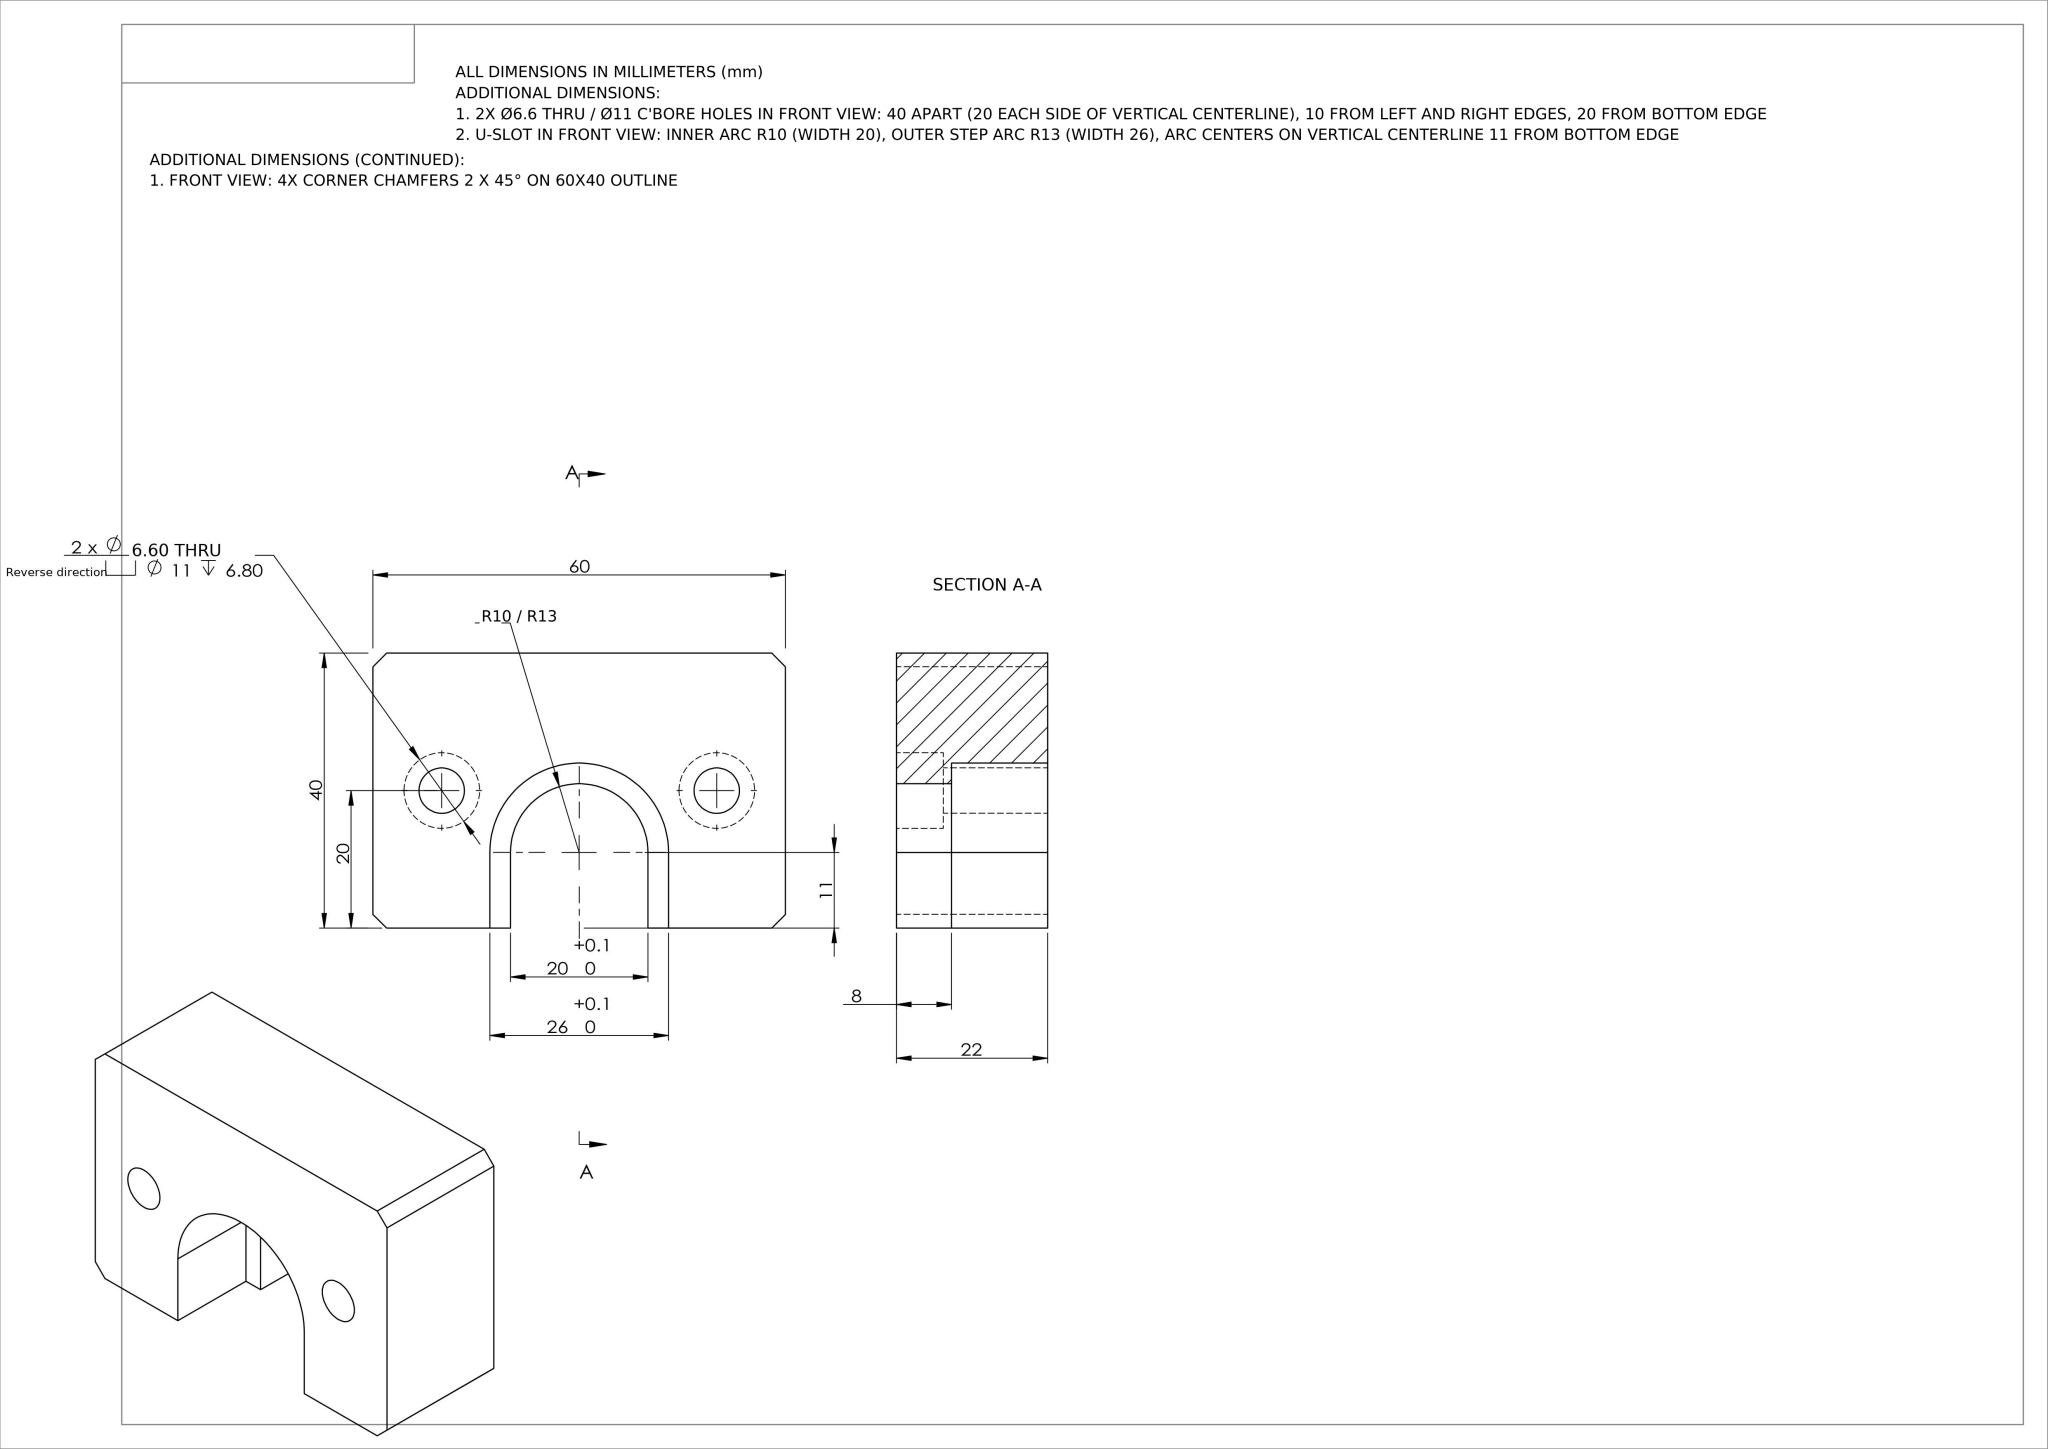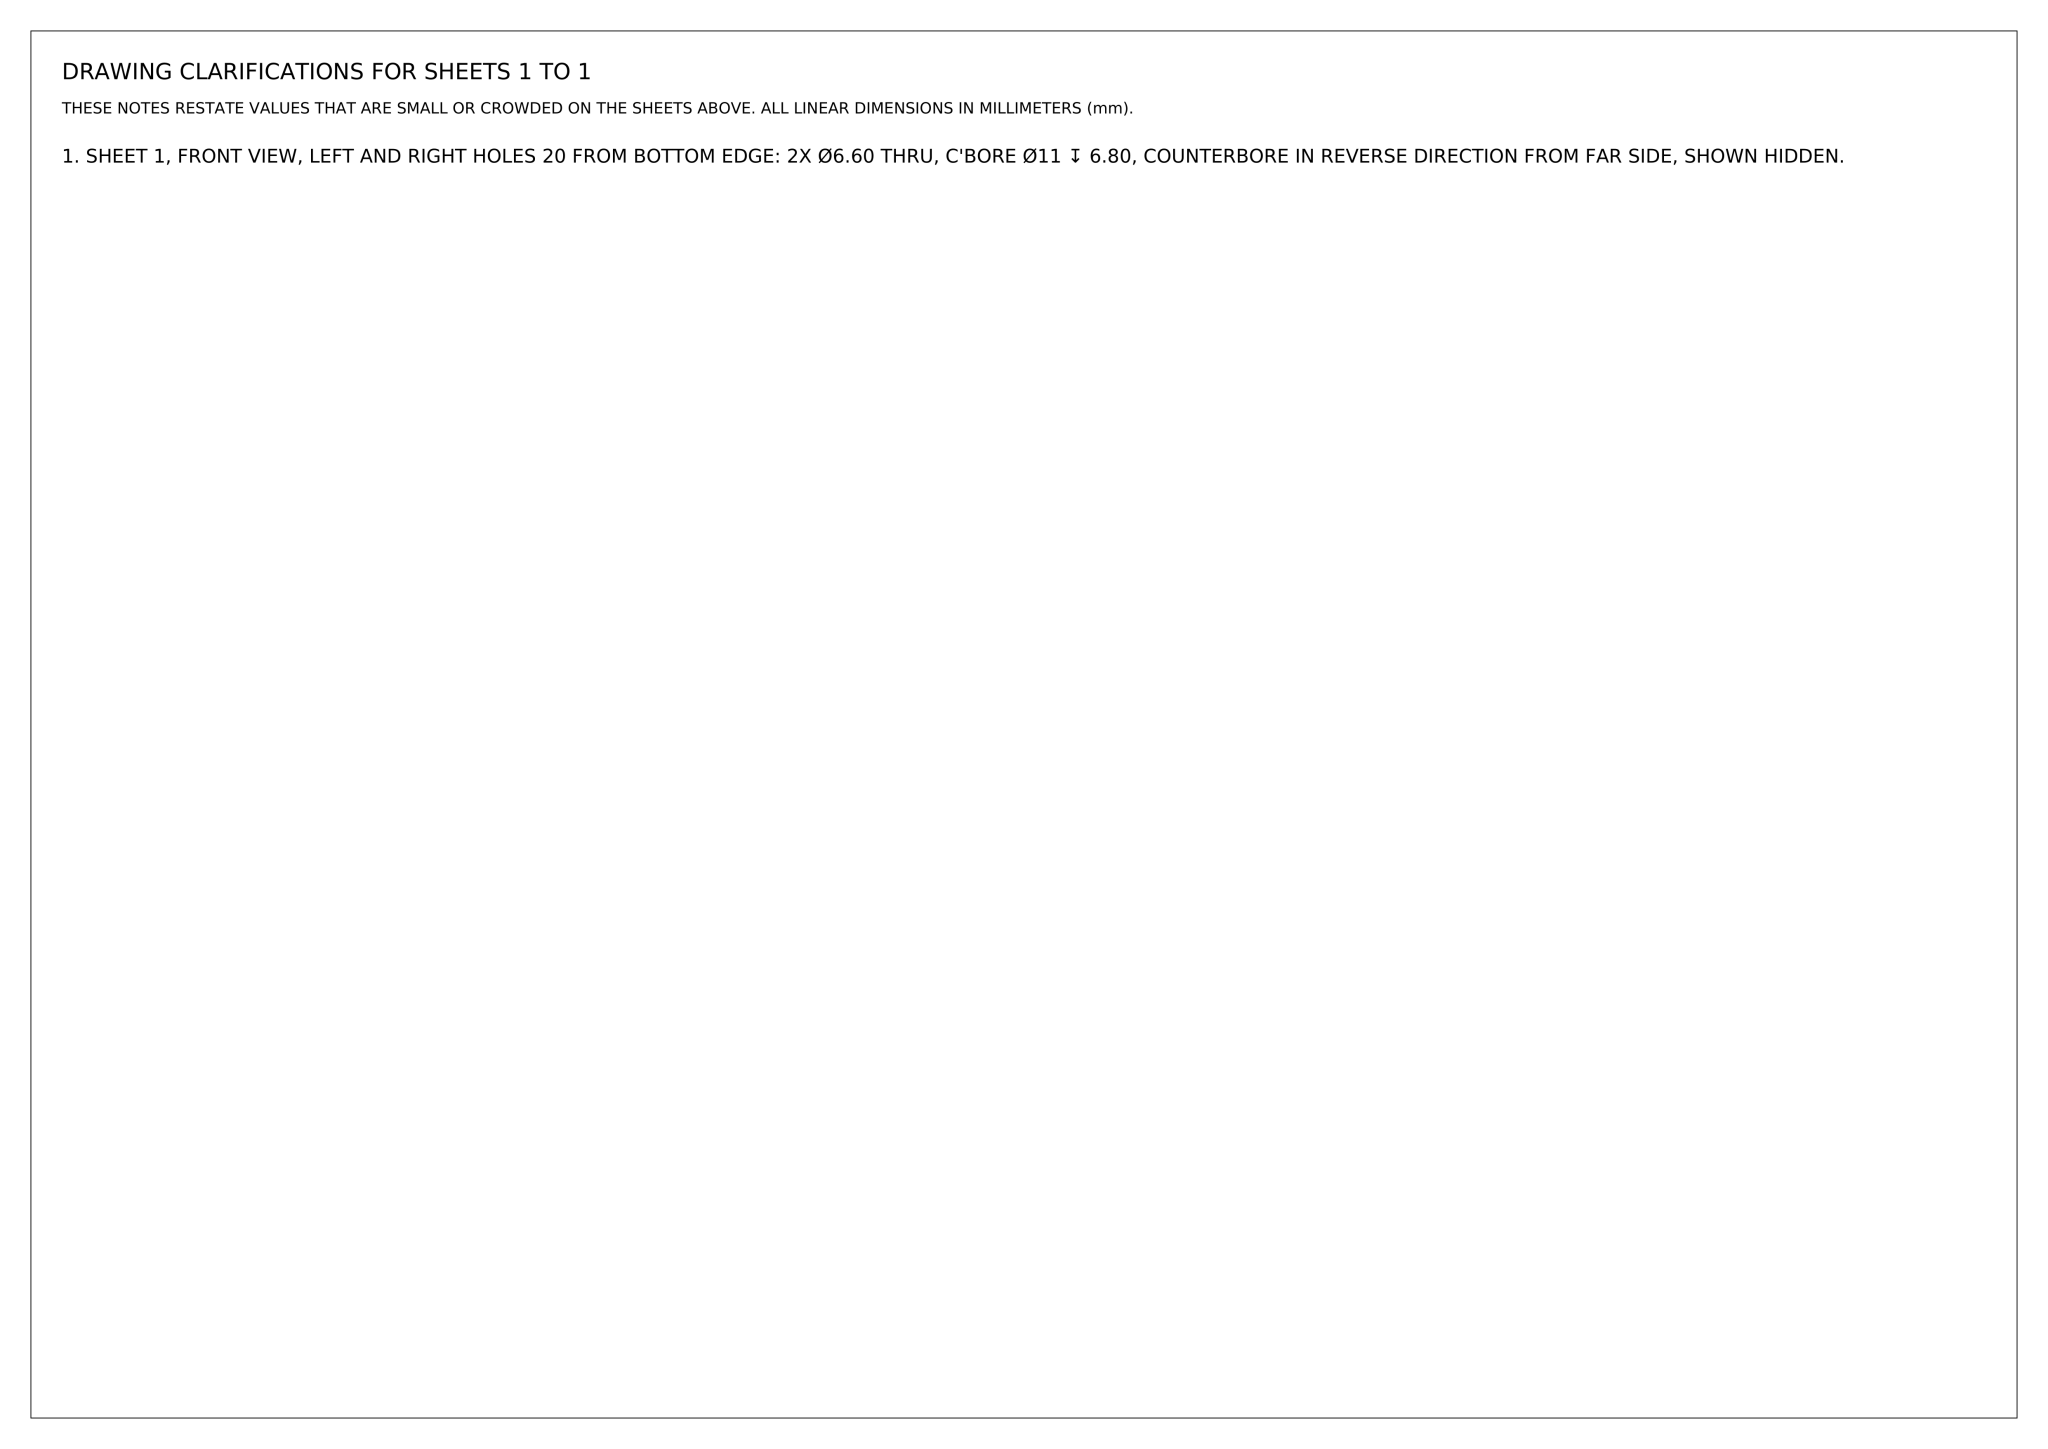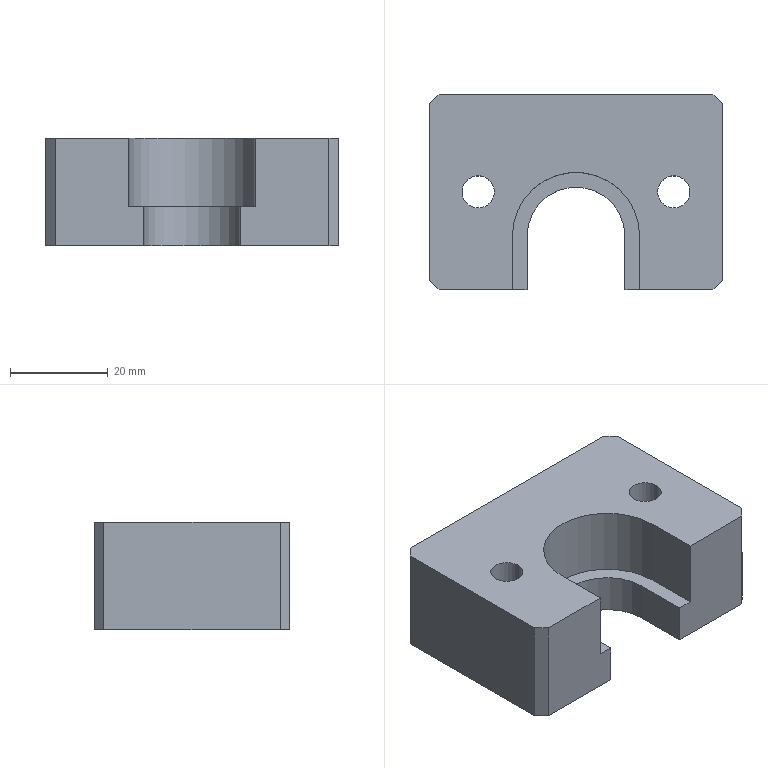Part | NX | mm | 1 solid | 28 faces | box 60 x 40 x 22 mm | volume 39554 mm3 | plane 18 | cylinder 10 | commonest cylinder face diameters 11 x4 6.6 x4 20 x1 26 x1
STEP:
#1=COLOUR_RGB('',0.6157,0.6431,0.6745);
#2=FILL_AREA_STYLE_COLOUR('',#1);
#3=FILL_AREA_STYLE('',(#2));
#4=SURFACE_STYLE_FILL_AREA(#3);
#5=SURFACE_SIDE_STYLE('',(#4));
#6=SURFACE_STYLE_USAGE(.BOTH.,#5);
#7=PRESENTATION_STYLE_ASSIGNMENT((#6));
#8=CARTESIAN_POINT('',(25.5,-0.,6.8));
#9=VERTEX_POINT('',#8);
#10=CARTESIAN_POINT('',(14.5,-0.,6.8));
#11=VERTEX_POINT('',#10);
#12=CARTESIAN_POINT('',(20.,-0.,6.8));
#13=DIRECTION('',(0.,0.,-1.));
#14=DIRECTION('',(-1.,0.,0.));
#15=AXIS2_PLACEMENT_3D('',#12,#13,#14);
#16=CIRCLE('',#15,5.5);
#17=EDGE_CURVE('',#9,#11,#16,.T.);
#18=ORIENTED_EDGE('',*,*,#17,.F.);
#19=CARTESIAN_POINT('',(25.5,-0.,0.));
#20=VERTEX_POINT('',#19);
#21=CARTESIAN_POINT('',(25.5,-0.,0.));
#22=DIRECTION('',(0.,0.,-1.));
#23=VECTOR('',#22,1000.);
#24=LINE('',#21,#23);
#25=EDGE_CURVE('',#9,#20,#24,.T.);
#26=ORIENTED_EDGE('',*,*,#25,.T.);
#27=CARTESIAN_POINT('',(14.5,-0.,0.));
#28=VERTEX_POINT('',#27);
#29=CARTESIAN_POINT('',(20.,-0.,0.));
#30=DIRECTION('',(0.,0.,-1.));
#31=DIRECTION('',(-1.,0.,0.));
#32=AXIS2_PLACEMENT_3D('',#29,#30,#31);
#33=CIRCLE('',#32,5.5);
#34=EDGE_CURVE('',#20,#28,#33,.T.);
#35=ORIENTED_EDGE('',*,*,#34,.T.);
#36=CARTESIAN_POINT('',(14.5,-0.,0.));
#37=DIRECTION('',(0.,0.,-1.));
#38=VECTOR('',#37,1000.);
#39=LINE('',#36,#38);
#40=EDGE_CURVE('',#11,#28,#39,.T.);
#41=ORIENTED_EDGE('',*,*,#40,.F.);
#42=EDGE_LOOP('',(#18,#26,#35,#41));
#43=FACE_OUTER_BOUND('',#42,.T.);
#44=CARTESIAN_POINT('',(20.,-0.,0.));
#45=DIRECTION('',(0.,0.,-1.));
#46=DIRECTION('',(-1.,0.,0.));
#47=AXIS2_PLACEMENT_3D('',#44,#45,#46);
#48=CYLINDRICAL_SURFACE('',#47,5.5);
#49=ADVANCED_FACE('',(#43),#48,.F.);
#50=CARTESIAN_POINT('',(23.3,-0.,22.));
#51=VERTEX_POINT('',#50);
#52=CARTESIAN_POINT('',(16.7,-0.,22.));
#53=VERTEX_POINT('',#52);
#54=CARTESIAN_POINT('',(20.,-0.,22.));
#55=DIRECTION('',(0.,0.,-1.));
#56=DIRECTION('',(-1.,0.,0.));
#57=AXIS2_PLACEMENT_3D('',#54,#55,#56);
#58=CIRCLE('',#57,3.3);
#59=EDGE_CURVE('',#51,#53,#58,.T.);
#60=ORIENTED_EDGE('',*,*,#59,.F.);
#61=CARTESIAN_POINT('',(23.3,-0.,6.8));
#62=VERTEX_POINT('',#61);
#63=CARTESIAN_POINT('',(23.3,-0.,0.));
#64=DIRECTION('',(0.,0.,-1.));
#65=VECTOR('',#64,1000.);
#66=LINE('',#63,#65);
#67=EDGE_CURVE('',#51,#62,#66,.T.);
#68=ORIENTED_EDGE('',*,*,#67,.T.);
#69=CARTESIAN_POINT('',(16.7,-0.,6.8));
#70=VERTEX_POINT('',#69);
#71=CARTESIAN_POINT('',(20.,-0.,6.8));
#72=DIRECTION('',(0.,0.,-1.));
#73=DIRECTION('',(-1.,0.,0.));
#74=AXIS2_PLACEMENT_3D('',#71,#72,#73);
#75=CIRCLE('',#74,3.3);
#76=EDGE_CURVE('',#62,#70,#75,.T.);
#77=ORIENTED_EDGE('',*,*,#76,.T.);
#78=CARTESIAN_POINT('',(16.7,-0.,0.));
#79=DIRECTION('',(0.,0.,-1.));
#80=VECTOR('',#79,1000.);
#81=LINE('',#78,#80);
#82=EDGE_CURVE('',#53,#70,#81,.T.);
#83=ORIENTED_EDGE('',*,*,#82,.F.);
#84=EDGE_LOOP('',(#60,#68,#77,#83));
#85=FACE_OUTER_BOUND('',#84,.T.);
#86=CARTESIAN_POINT('',(20.,-0.,0.));
#87=DIRECTION('',(0.,0.,-1.));
#88=DIRECTION('',(-1.,0.,0.));
#89=AXIS2_PLACEMENT_3D('',#86,#87,#88);
#90=CYLINDRICAL_SURFACE('',#89,3.3);
#91=ADVANCED_FACE('',(#85),#90,.F.);
#92=CARTESIAN_POINT('',(-14.5,-0.,6.8));
#93=VERTEX_POINT('',#92);
#94=CARTESIAN_POINT('',(-25.5,-0.,6.8));
#95=VERTEX_POINT('',#94);
#96=CARTESIAN_POINT('',(-20.,-0.,6.8));
#97=DIRECTION('',(0.,0.,-1.));
#98=DIRECTION('',(-1.,0.,0.));
#99=AXIS2_PLACEMENT_3D('',#96,#97,#98);
#100=CIRCLE('',#99,5.5);
#101=EDGE_CURVE('',#93,#95,#100,.T.);
#102=ORIENTED_EDGE('',*,*,#101,.F.);
#103=CARTESIAN_POINT('',(-14.5,-0.,0.));
#104=VERTEX_POINT('',#103);
#105=CARTESIAN_POINT('',(-14.5,-0.,0.));
#106=DIRECTION('',(0.,0.,-1.));
#107=VECTOR('',#106,1000.);
#108=LINE('',#105,#107);
#109=EDGE_CURVE('',#93,#104,#108,.T.);
#110=ORIENTED_EDGE('',*,*,#109,.T.);
#111=CARTESIAN_POINT('',(-25.5,-0.,0.));
#112=VERTEX_POINT('',#111);
#113=CARTESIAN_POINT('',(-20.,-0.,0.));
#114=DIRECTION('',(0.,0.,-1.));
#115=DIRECTION('',(-1.,0.,0.));
#116=AXIS2_PLACEMENT_3D('',#113,#114,#115);
#117=CIRCLE('',#116,5.5);
#118=EDGE_CURVE('',#104,#112,#117,.T.);
#119=ORIENTED_EDGE('',*,*,#118,.T.);
#120=CARTESIAN_POINT('',(-25.5,-0.,0.));
#121=DIRECTION('',(0.,0.,-1.));
#122=VECTOR('',#121,1000.);
#123=LINE('',#120,#122);
#124=EDGE_CURVE('',#95,#112,#123,.T.);
#125=ORIENTED_EDGE('',*,*,#124,.F.);
#126=EDGE_LOOP('',(#102,#110,#119,#125));
#127=FACE_OUTER_BOUND('',#126,.T.);
#128=CARTESIAN_POINT('',(-20.,-0.,0.));
#129=DIRECTION('',(0.,0.,-1.));
#130=DIRECTION('',(-1.,0.,0.));
#131=AXIS2_PLACEMENT_3D('',#128,#129,#130);
#132=CYLINDRICAL_SURFACE('',#131,5.5);
#133=ADVANCED_FACE('',(#127),#132,.F.);
#134=CARTESIAN_POINT('',(-16.7,-0.,22.));
#135=VERTEX_POINT('',#134);
#136=CARTESIAN_POINT('',(-23.3,-0.,22.));
#137=VERTEX_POINT('',#136);
#138=CARTESIAN_POINT('',(-20.,-0.,22.));
#139=DIRECTION('',(0.,0.,-1.));
#140=DIRECTION('',(-1.,0.,0.));
#141=AXIS2_PLACEMENT_3D('',#138,#139,#140);
#142=CIRCLE('',#141,3.3);
#143=EDGE_CURVE('',#135,#137,#142,.T.);
#144=ORIENTED_EDGE('',*,*,#143,.F.);
#145=CARTESIAN_POINT('',(-16.7,-0.,6.8));
#146=VERTEX_POINT('',#145);
#147=CARTESIAN_POINT('',(-16.7,-0.,0.));
#148=DIRECTION('',(0.,0.,-1.));
#149=VECTOR('',#148,1000.);
#150=LINE('',#147,#149);
#151=EDGE_CURVE('',#135,#146,#150,.T.);
#152=ORIENTED_EDGE('',*,*,#151,.T.);
#153=CARTESIAN_POINT('',(-23.3,-0.,6.8));
#154=VERTEX_POINT('',#153);
#155=CARTESIAN_POINT('',(-20.,-0.,6.8));
#156=DIRECTION('',(0.,0.,-1.));
#157=DIRECTION('',(-1.,0.,0.));
#158=AXIS2_PLACEMENT_3D('',#155,#156,#157);
#159=CIRCLE('',#158,3.3);
#160=EDGE_CURVE('',#146,#154,#159,.T.);
#161=ORIENTED_EDGE('',*,*,#160,.T.);
#162=CARTESIAN_POINT('',(-23.3,-0.,0.));
#163=DIRECTION('',(0.,0.,-1.));
#164=VECTOR('',#163,1000.);
#165=LINE('',#162,#164);
#166=EDGE_CURVE('',#137,#154,#165,.T.);
#167=ORIENTED_EDGE('',*,*,#166,.F.);
#168=EDGE_LOOP('',(#144,#152,#161,#167));
#169=FACE_OUTER_BOUND('',#168,.T.);
#170=CARTESIAN_POINT('',(-20.,-0.,0.));
#171=DIRECTION('',(0.,0.,-1.));
#172=DIRECTION('',(-1.,0.,0.));
#173=AXIS2_PLACEMENT_3D('',#170,#171,#172);
#174=CYLINDRICAL_SURFACE('',#173,3.3);
#175=ADVANCED_FACE('',(#169),#174,.F.);
#176=CARTESIAN_POINT('',(-10.,-20.,8.));
#177=VERTEX_POINT('',#176);
#178=CARTESIAN_POINT('',(-10.,-9.,8.));
#179=VERTEX_POINT('',#178);
#180=CARTESIAN_POINT('',(-10.,-20.,8.));
#181=DIRECTION('',(0.,1.,0.));
#182=VECTOR('',#181,1000.);
#183=LINE('',#180,#182);
#184=EDGE_CURVE('',#177,#179,#183,.T.);
#185=ORIENTED_EDGE('',*,*,#184,.F.);
#186=CARTESIAN_POINT('',(-10.,-20.,0.));
#187=VERTEX_POINT('',#186);
#188=CARTESIAN_POINT('',(-10.,-20.,0.));
#189=DIRECTION('',(0.,0.,1.));
#190=VECTOR('',#189,1000.);
#191=LINE('',#188,#190);
#192=EDGE_CURVE('',#187,#177,#191,.T.);
#193=ORIENTED_EDGE('',*,*,#192,.F.);
#194=CARTESIAN_POINT('',(-10.,-9.,0.));
#195=VERTEX_POINT('',#194);
#196=CARTESIAN_POINT('',(-10.,-20.,0.));
#197=DIRECTION('',(0.,-1.,0.));
#198=VECTOR('',#197,1000.);
#199=LINE('',#196,#198);
#200=EDGE_CURVE('',#195,#187,#199,.T.);
#201=ORIENTED_EDGE('',*,*,#200,.F.);
#202=CARTESIAN_POINT('',(-10.,-9.,0.));
#203=DIRECTION('',(0.,0.,1.));
#204=VECTOR('',#203,1000.);
#205=LINE('',#202,#204);
#206=EDGE_CURVE('',#195,#179,#205,.T.);
#207=ORIENTED_EDGE('',*,*,#206,.T.);
#208=EDGE_LOOP('',(#185,#193,#201,#207));
#209=FACE_OUTER_BOUND('',#208,.T.);
#210=CARTESIAN_POINT('',(-10.,-20.,0.));
#211=DIRECTION('',(-1.,0.,0.));
#212=DIRECTION('',(0.,0.,1.));
#213=AXIS2_PLACEMENT_3D('',#210,#211,#212);
#214=PLANE('',#213);
#215=ADVANCED_FACE('',(#209),#214,.F.);
#216=CARTESIAN_POINT('',(10.,-9.,8.));
#217=VERTEX_POINT('',#216);
#218=CARTESIAN_POINT('',(0.,-9.,8.));
#219=DIRECTION('',(0.,0.,-1.));
#220=DIRECTION('',(1.,0.,0.));
#221=AXIS2_PLACEMENT_3D('',#218,#219,#220);
#222=CIRCLE('',#221,10.);
#223=EDGE_CURVE('',#179,#217,#222,.T.);
#224=ORIENTED_EDGE('',*,*,#223,.F.);
#225=ORIENTED_EDGE('',*,*,#206,.F.);
#226=CARTESIAN_POINT('',(10.,-9.,0.));
#227=VERTEX_POINT('',#226);
#228=CARTESIAN_POINT('',(0.,-9.,0.));
#229=DIRECTION('',(0.,0.,1.));
#230=DIRECTION('',(1.,0.,0.));
#231=AXIS2_PLACEMENT_3D('',#228,#229,#230);
#232=CIRCLE('',#231,10.);
#233=EDGE_CURVE('',#227,#195,#232,.T.);
#234=ORIENTED_EDGE('',*,*,#233,.F.);
#235=CARTESIAN_POINT('',(10.,-9.,0.));
#236=DIRECTION('',(0.,0.,1.));
#237=VECTOR('',#236,1000.);
#238=LINE('',#235,#237);
#239=EDGE_CURVE('',#227,#217,#238,.T.);
#240=ORIENTED_EDGE('',*,*,#239,.T.);
#241=EDGE_LOOP('',(#224,#225,#234,#240));
#242=FACE_OUTER_BOUND('',#241,.T.);
#243=CARTESIAN_POINT('',(0.,-9.,0.));
#244=DIRECTION('',(0.,0.,1.));
#245=DIRECTION('',(1.,0.,0.));
#246=AXIS2_PLACEMENT_3D('',#243,#244,#245);
#247=CYLINDRICAL_SURFACE('',#246,10.);
#248=ADVANCED_FACE('',(#242),#247,.F.);
#249=CARTESIAN_POINT('',(10.,-20.,8.));
#250=VERTEX_POINT('',#249);
#251=CARTESIAN_POINT('',(10.,-20.,8.));
#252=DIRECTION('',(0.,-1.,0.));
#253=VECTOR('',#252,1000.);
#254=LINE('',#251,#253);
#255=EDGE_CURVE('',#217,#250,#254,.T.);
#256=ORIENTED_EDGE('',*,*,#255,.F.);
#257=ORIENTED_EDGE('',*,*,#239,.F.);
#258=CARTESIAN_POINT('',(10.,-20.,0.));
#259=VERTEX_POINT('',#258);
#260=CARTESIAN_POINT('',(10.,-20.,0.));
#261=DIRECTION('',(0.,1.,0.));
#262=VECTOR('',#261,1000.);
#263=LINE('',#260,#262);
#264=EDGE_CURVE('',#259,#227,#263,.T.);
#265=ORIENTED_EDGE('',*,*,#264,.F.);
#266=CARTESIAN_POINT('',(10.,-20.,0.));
#267=DIRECTION('',(0.,0.,1.));
#268=VECTOR('',#267,1000.);
#269=LINE('',#266,#268);
#270=EDGE_CURVE('',#259,#250,#269,.T.);
#271=ORIENTED_EDGE('',*,*,#270,.T.);
#272=EDGE_LOOP('',(#256,#257,#265,#271));
#273=FACE_OUTER_BOUND('',#272,.T.);
#274=CARTESIAN_POINT('',(10.,-20.,0.));
#275=DIRECTION('',(1.,0.,0.));
#276=DIRECTION('',(0.,0.,-1.));
#277=AXIS2_PLACEMENT_3D('',#274,#275,#276);
#278=PLANE('',#277);
#279=ADVANCED_FACE('',(#273),#278,.F.);
#280=CARTESIAN_POINT('',(-28.,-20.,22.));
#281=VERTEX_POINT('',#280);
#282=CARTESIAN_POINT('',(-13.,-20.,22.));
#283=VERTEX_POINT('',#282);
#284=CARTESIAN_POINT('',(-30.,-20.,22.));
#285=DIRECTION('',(1.,0.,0.));
#286=VECTOR('',#285,1000.);
#287=LINE('',#284,#286);
#288=EDGE_CURVE('',#281,#283,#287,.T.);
#289=ORIENTED_EDGE('',*,*,#288,.F.);
#290=CARTESIAN_POINT('',(-28.,-20.,0.));
#291=VERTEX_POINT('',#290);
#292=CARTESIAN_POINT('',(-28.,-20.,22.));
#293=DIRECTION('',(0.,0.,-1.));
#294=VECTOR('',#293,1000.);
#295=LINE('',#292,#294);
#296=EDGE_CURVE('',#281,#291,#295,.T.);
#297=ORIENTED_EDGE('',*,*,#296,.T.);
#298=CARTESIAN_POINT('',(-30.,-20.,0.));
#299=DIRECTION('',(1.,0.,0.));
#300=VECTOR('',#299,1000.);
#301=LINE('',#298,#300);
#302=EDGE_CURVE('',#291,#187,#301,.T.);
#303=ORIENTED_EDGE('',*,*,#302,.T.);
#304=ORIENTED_EDGE('',*,*,#192,.T.);
#305=CARTESIAN_POINT('',(-13.,-20.,8.));
#306=VERTEX_POINT('',#305);
#307=CARTESIAN_POINT('',(-13.,-20.,8.));
#308=DIRECTION('',(1.,0.,0.));
#309=VECTOR('',#308,1000.);
#310=LINE('',#307,#309);
#311=EDGE_CURVE('',#306,#177,#310,.T.);
#312=ORIENTED_EDGE('',*,*,#311,.F.);
#313=CARTESIAN_POINT('',(-13.,-20.,8.));
#314=DIRECTION('',(0.,0.,1.));
#315=VECTOR('',#314,1000.);
#316=LINE('',#313,#315);
#317=EDGE_CURVE('',#306,#283,#316,.T.);
#318=ORIENTED_EDGE('',*,*,#317,.T.);
#319=EDGE_LOOP('',(#289,#297,#303,#304,#312,#318));
#320=FACE_OUTER_BOUND('',#319,.T.);
#321=CARTESIAN_POINT('',(-30.,-20.,22.));
#322=DIRECTION('',(0.,1.,0.));
#323=DIRECTION('',(0.,0.,1.));
#324=AXIS2_PLACEMENT_3D('',#321,#322,#323);
#325=PLANE('',#324);
#326=ADVANCED_FACE('',(#320),#325,.F.);
#327=CARTESIAN_POINT('',(30.,-18.,22.));
#328=VERTEX_POINT('',#327);
#329=CARTESIAN_POINT('',(30.,18.,22.));
#330=VERTEX_POINT('',#329);
#331=CARTESIAN_POINT('',(30.,-20.,22.));
#332=DIRECTION('',(0.,1.,0.));
#333=VECTOR('',#332,1000.);
#334=LINE('',#331,#333);
#335=EDGE_CURVE('',#328,#330,#334,.T.);
#336=ORIENTED_EDGE('',*,*,#335,.F.);
#337=CARTESIAN_POINT('',(30.,-18.,0.));
#338=VERTEX_POINT('',#337);
#339=CARTESIAN_POINT('',(30.,-18.,22.));
#340=DIRECTION('',(0.,0.,-1.));
#341=VECTOR('',#340,1000.);
#342=LINE('',#339,#341);
#343=EDGE_CURVE('',#328,#338,#342,.T.);
#344=ORIENTED_EDGE('',*,*,#343,.T.);
#345=CARTESIAN_POINT('',(30.,18.,0.));
#346=VERTEX_POINT('',#345);
#347=CARTESIAN_POINT('',(30.,-20.,0.));
#348=DIRECTION('',(0.,1.,0.));
#349=VECTOR('',#348,1000.);
#350=LINE('',#347,#349);
#351=EDGE_CURVE('',#338,#346,#350,.T.);
#352=ORIENTED_EDGE('',*,*,#351,.T.);
#353=CARTESIAN_POINT('',(30.,18.,22.));
#354=DIRECTION('',(0.,0.,1.));
#355=VECTOR('',#354,1000.);
#356=LINE('',#353,#355);
#357=EDGE_CURVE('',#346,#330,#356,.T.);
#358=ORIENTED_EDGE('',*,*,#357,.T.);
#359=EDGE_LOOP('',(#336,#344,#352,#358));
#360=FACE_OUTER_BOUND('',#359,.T.);
#361=CARTESIAN_POINT('',(30.,-20.,22.));
#362=DIRECTION('',(-1.,0.,0.));
#363=DIRECTION('',(0.,0.,1.));
#364=AXIS2_PLACEMENT_3D('',#361,#362,#363);
#365=PLANE('',#364);
#366=ADVANCED_FACE('',(#360),#365,.F.);
#367=CARTESIAN_POINT('',(28.,20.,0.));
#368=VERTEX_POINT('',#367);
#369=CARTESIAN_POINT('',(-28.,20.,0.));
#370=VERTEX_POINT('',#369);
#371=CARTESIAN_POINT('',(-30.,20.,0.));
#372=DIRECTION('',(-1.,0.,0.));
#373=VECTOR('',#372,1000.);
#374=LINE('',#371,#373);
#375=EDGE_CURVE('',#368,#370,#374,.T.);
#376=ORIENTED_EDGE('',*,*,#375,.T.);
#377=CARTESIAN_POINT('',(-28.,20.,22.));
#378=VERTEX_POINT('',#377);
#379=CARTESIAN_POINT('',(-28.,20.,22.));
#380=DIRECTION('',(0.,0.,1.));
#381=VECTOR('',#380,1000.);
#382=LINE('',#379,#381);
#383=EDGE_CURVE('',#370,#378,#382,.T.);
#384=ORIENTED_EDGE('',*,*,#383,.T.);
#385=CARTESIAN_POINT('',(28.,20.,22.));
#386=VERTEX_POINT('',#385);
#387=CARTESIAN_POINT('',(-30.,20.,22.));
#388=DIRECTION('',(-1.,0.,0.));
#389=VECTOR('',#388,1000.);
#390=LINE('',#387,#389);
#391=EDGE_CURVE('',#386,#378,#390,.T.);
#392=ORIENTED_EDGE('',*,*,#391,.F.);
#393=CARTESIAN_POINT('',(28.,20.,22.));
#394=DIRECTION('',(0.,0.,-1.));
#395=VECTOR('',#394,1000.);
#396=LINE('',#393,#395);
#397=EDGE_CURVE('',#386,#368,#396,.T.);
#398=ORIENTED_EDGE('',*,*,#397,.T.);
#399=EDGE_LOOP('',(#376,#384,#392,#398));
#400=FACE_OUTER_BOUND('',#399,.T.);
#401=CARTESIAN_POINT('',(-30.,20.,22.));
#402=DIRECTION('',(0.,-1.,0.));
#403=DIRECTION('',(0.,0.,-1.));
#404=AXIS2_PLACEMENT_3D('',#401,#402,#403);
#405=PLANE('',#404);
#406=ADVANCED_FACE('',(#400),#405,.F.);
#407=CARTESIAN_POINT('',(-30.,18.,0.));
#408=VERTEX_POINT('',#407);
#409=CARTESIAN_POINT('',(-30.,-18.,0.));
#410=VERTEX_POINT('',#409);
#411=CARTESIAN_POINT('',(-30.,-20.,0.));
#412=DIRECTION('',(0.,-1.,0.));
#413=VECTOR('',#412,1000.);
#414=LINE('',#411,#413);
#415=EDGE_CURVE('',#408,#410,#414,.T.);
#416=ORIENTED_EDGE('',*,*,#415,.T.);
#417=CARTESIAN_POINT('',(-30.,-18.,22.));
#418=VERTEX_POINT('',#417);
#419=CARTESIAN_POINT('',(-30.,-18.,22.));
#420=DIRECTION('',(0.,0.,1.));
#421=VECTOR('',#420,1000.);
#422=LINE('',#419,#421);
#423=EDGE_CURVE('',#410,#418,#422,.T.);
#424=ORIENTED_EDGE('',*,*,#423,.T.);
#425=CARTESIAN_POINT('',(-30.,18.,22.));
#426=VERTEX_POINT('',#425);
#427=CARTESIAN_POINT('',(-30.,-20.,22.));
#428=DIRECTION('',(0.,-1.,0.));
#429=VECTOR('',#428,1000.);
#430=LINE('',#427,#429);
#431=EDGE_CURVE('',#426,#418,#430,.T.);
#432=ORIENTED_EDGE('',*,*,#431,.F.);
#433=CARTESIAN_POINT('',(-30.,18.,22.));
#434=DIRECTION('',(0.,0.,-1.));
#435=VECTOR('',#434,1000.);
#436=LINE('',#433,#435);
#437=EDGE_CURVE('',#426,#408,#436,.T.);
#438=ORIENTED_EDGE('',*,*,#437,.T.);
#439=EDGE_LOOP('',(#416,#424,#432,#438));
#440=FACE_OUTER_BOUND('',#439,.T.);
#441=CARTESIAN_POINT('',(-30.,-20.,22.));
#442=DIRECTION('',(1.,0.,0.));
#443=DIRECTION('',(0.,0.,-1.));
#444=AXIS2_PLACEMENT_3D('',#441,#442,#443);
#445=PLANE('',#444);
#446=ADVANCED_FACE('',(#440),#445,.F.);
#447=CARTESIAN_POINT('',(28.,-20.,0.));
#448=VERTEX_POINT('',#447);
#449=CARTESIAN_POINT('',(-30.,-20.,0.));
#450=DIRECTION('',(1.,0.,0.));
#451=VECTOR('',#450,1000.);
#452=LINE('',#449,#451);
#453=EDGE_CURVE('',#259,#448,#452,.T.);
#454=ORIENTED_EDGE('',*,*,#453,.T.);
#455=CARTESIAN_POINT('',(28.,-20.,22.));
#456=VERTEX_POINT('',#455);
#457=CARTESIAN_POINT('',(28.,-20.,22.));
#458=DIRECTION('',(0.,0.,1.));
#459=VECTOR('',#458,1000.);
#460=LINE('',#457,#459);
#461=EDGE_CURVE('',#448,#456,#460,.T.);
#462=ORIENTED_EDGE('',*,*,#461,.T.);
#463=CARTESIAN_POINT('',(13.,-20.,22.));
#464=VERTEX_POINT('',#463);
#465=CARTESIAN_POINT('',(-30.,-20.,22.));
#466=DIRECTION('',(1.,0.,0.));
#467=VECTOR('',#466,1000.);
#468=LINE('',#465,#467);
#469=EDGE_CURVE('',#464,#456,#468,.T.);
#470=ORIENTED_EDGE('',*,*,#469,.F.);
#471=CARTESIAN_POINT('',(13.,-20.,8.));
#472=VERTEX_POINT('',#471);
#473=CARTESIAN_POINT('',(13.,-20.,8.));
#474=DIRECTION('',(0.,0.,1.));
#475=VECTOR('',#474,1000.);
#476=LINE('',#473,#475);
#477=EDGE_CURVE('',#472,#464,#476,.T.);
#478=ORIENTED_EDGE('',*,*,#477,.F.);
#479=CARTESIAN_POINT('',(-13.,-20.,8.));
#480=DIRECTION('',(1.,0.,0.));
#481=VECTOR('',#480,1000.);
#482=LINE('',#479,#481);
#483=EDGE_CURVE('',#250,#472,#482,.T.);
#484=ORIENTED_EDGE('',*,*,#483,.F.);
#485=ORIENTED_EDGE('',*,*,#270,.F.);
#486=EDGE_LOOP('',(#454,#462,#470,#478,#484,#485));
#487=FACE_OUTER_BOUND('',#486,.T.);
#488=CARTESIAN_POINT('',(-30.,-20.,22.));
#489=DIRECTION('',(0.,1.,0.));
#490=DIRECTION('',(0.,0.,1.));
#491=AXIS2_PLACEMENT_3D('',#488,#489,#490);
#492=PLANE('',#491);
#493=ADVANCED_FACE('',(#487),#492,.F.);
#494=CARTESIAN_POINT('',(20.,-0.,22.));
#495=DIRECTION('',(0.,0.,-1.));
#496=DIRECTION('',(-1.,0.,0.));
#497=AXIS2_PLACEMENT_3D('',#494,#495,#496);
#498=CIRCLE('',#497,3.3);
#499=EDGE_CURVE('',#53,#51,#498,.T.);
#500=ORIENTED_EDGE('',*,*,#499,.T.);
#501=ORIENTED_EDGE('',*,*,#59,.T.);
#502=EDGE_LOOP('',(#500,#501));
#503=FACE_BOUND('',#502,.T.);
#504=CARTESIAN_POINT('',(-20.,-0.,22.));
#505=DIRECTION('',(0.,0.,-1.));
#506=DIRECTION('',(-1.,0.,0.));
#507=AXIS2_PLACEMENT_3D('',#504,#505,#506);
#508=CIRCLE('',#507,3.3);
#509=EDGE_CURVE('',#137,#135,#508,.T.);
#510=ORIENTED_EDGE('',*,*,#509,.T.);
#511=ORIENTED_EDGE('',*,*,#143,.T.);
#512=EDGE_LOOP('',(#510,#511));
#513=FACE_BOUND('',#512,.T.);
#514=ORIENTED_EDGE('',*,*,#469,.T.);
#515=CARTESIAN_POINT('',(30.,-18.,22.));
#516=DIRECTION('',(0.7071,0.7071,0.));
#517=VECTOR('',#516,1000.);
#518=LINE('',#515,#517);
#519=EDGE_CURVE('',#456,#328,#518,.T.);
#520=ORIENTED_EDGE('',*,*,#519,.T.);
#521=ORIENTED_EDGE('',*,*,#335,.T.);
#522=CARTESIAN_POINT('',(28.,20.,22.));
#523=DIRECTION('',(-0.7071,0.7071,0.));
#524=VECTOR('',#523,1000.);
#525=LINE('',#522,#524);
#526=EDGE_CURVE('',#330,#386,#525,.T.);
#527=ORIENTED_EDGE('',*,*,#526,.T.);
#528=ORIENTED_EDGE('',*,*,#391,.T.);
#529=CARTESIAN_POINT('',(-30.,18.,22.));
#530=DIRECTION('',(-0.7071,-0.7071,0.));
#531=VECTOR('',#530,1000.);
#532=LINE('',#529,#531);
#533=EDGE_CURVE('',#378,#426,#532,.T.);
#534=ORIENTED_EDGE('',*,*,#533,.T.);
#535=ORIENTED_EDGE('',*,*,#431,.T.);
#536=CARTESIAN_POINT('',(-28.,-20.,22.));
#537=DIRECTION('',(0.7071,-0.7071,0.));
#538=VECTOR('',#537,1000.);
#539=LINE('',#536,#538);
#540=EDGE_CURVE('',#418,#281,#539,.T.);
#541=ORIENTED_EDGE('',*,*,#540,.T.);
#542=ORIENTED_EDGE('',*,*,#288,.T.);
#543=CARTESIAN_POINT('',(-13.,-9.,22.));
#544=VERTEX_POINT('',#543);
#545=CARTESIAN_POINT('',(-13.,-9.,22.));
#546=DIRECTION('',(0.,-1.,0.));
#547=VECTOR('',#546,1000.);
#548=LINE('',#545,#547);
#549=EDGE_CURVE('',#544,#283,#548,.T.);
#550=ORIENTED_EDGE('',*,*,#549,.F.);
#551=CARTESIAN_POINT('',(13.,-9.,22.));
#552=VERTEX_POINT('',#551);
#553=CARTESIAN_POINT('',(0.,-9.,22.));
#554=DIRECTION('',(0.,0.,1.));
#555=DIRECTION('',(1.,0.,0.));
#556=AXIS2_PLACEMENT_3D('',#553,#554,#555);
#557=CIRCLE('',#556,13.);
#558=EDGE_CURVE('',#552,#544,#557,.T.);
#559=ORIENTED_EDGE('',*,*,#558,.F.);
#560=CARTESIAN_POINT('',(13.,-20.,22.));
#561=DIRECTION('',(0.,1.,0.));
#562=VECTOR('',#561,1000.);
#563=LINE('',#560,#562);
#564=EDGE_CURVE('',#464,#552,#563,.T.);
#565=ORIENTED_EDGE('',*,*,#564,.F.);
#566=EDGE_LOOP('',(#514,#520,#521,#527,#528,#534,#535,#541,#542,#550,#559,#565));
#567=FACE_OUTER_BOUND('',#566,.T.);
#568=CARTESIAN_POINT('',(30.,20.,22.));
#569=DIRECTION('',(0.,0.,-1.));
#570=DIRECTION('',(-1.,0.,0.));
#571=AXIS2_PLACEMENT_3D('',#568,#569,#570);
#572=PLANE('',#571);
#573=ADVANCED_FACE('',(#503,#513,#567),#572,.F.);
#574=CARTESIAN_POINT('',(20.,-0.,0.));
#575=DIRECTION('',(0.,0.,-1.));
#576=DIRECTION('',(-1.,0.,0.));
#577=AXIS2_PLACEMENT_3D('',#574,#575,#576);
#578=CIRCLE('',#577,5.5);
#579=EDGE_CURVE('',#28,#20,#578,.T.);
#580=ORIENTED_EDGE('',*,*,#579,.F.);
#581=ORIENTED_EDGE('',*,*,#34,.F.);
#582=EDGE_LOOP('',(#580,#581));
#583=FACE_BOUND('',#582,.T.);
#584=CARTESIAN_POINT('',(-20.,-0.,0.));
#585=DIRECTION('',(0.,0.,-1.));
#586=DIRECTION('',(-1.,0.,0.));
#587=AXIS2_PLACEMENT_3D('',#584,#585,#586);
#588=CIRCLE('',#587,5.5);
#589=EDGE_CURVE('',#112,#104,#588,.T.);
#590=ORIENTED_EDGE('',*,*,#589,.F.);
#591=ORIENTED_EDGE('',*,*,#118,.F.);
#592=EDGE_LOOP('',(#590,#591));
#593=FACE_BOUND('',#592,.T.);
#594=ORIENTED_EDGE('',*,*,#351,.F.);
#595=CARTESIAN_POINT('',(49.,1.,0.));
#596=DIRECTION('',(-0.7071,-0.7071,0.));
#597=VECTOR('',#596,1000.);
#598=LINE('',#595,#597);
#599=EDGE_CURVE('',#338,#448,#598,.T.);
#600=ORIENTED_EDGE('',*,*,#599,.T.);
#601=ORIENTED_EDGE('',*,*,#453,.F.);
#602=ORIENTED_EDGE('',*,*,#264,.T.);
#603=ORIENTED_EDGE('',*,*,#233,.T.);
#604=ORIENTED_EDGE('',*,*,#200,.T.);
#605=ORIENTED_EDGE('',*,*,#302,.F.);
#606=CARTESIAN_POINT('',(-19.,-29.,0.));
#607=DIRECTION('',(-0.7071,0.7071,0.));
#608=VECTOR('',#607,1000.);
#609=LINE('',#606,#608);
#610=EDGE_CURVE('',#291,#410,#609,.T.);
#611=ORIENTED_EDGE('',*,*,#610,.T.);
#612=ORIENTED_EDGE('',*,*,#415,.F.);
#613=CARTESIAN_POINT('',(1.,49.,0.));
#614=DIRECTION('',(0.7071,0.7071,0.));
#615=VECTOR('',#614,1000.);
#616=LINE('',#613,#615);
#617=EDGE_CURVE('',#408,#370,#616,.T.);
#618=ORIENTED_EDGE('',*,*,#617,.T.);
#619=ORIENTED_EDGE('',*,*,#375,.F.);
#620=CARTESIAN_POINT('',(29.,19.,0.));
#621=DIRECTION('',(0.7071,-0.7071,0.));
#622=VECTOR('',#621,1000.);
#623=LINE('',#620,#622);
#624=EDGE_CURVE('',#368,#346,#623,.T.);
#625=ORIENTED_EDGE('',*,*,#624,.T.);
#626=EDGE_LOOP('',(#594,#600,#601,#602,#603,#604,#605,#611,#612,#618,#619,#625));
#627=FACE_OUTER_BOUND('',#626,.T.);
#628=CARTESIAN_POINT('',(30.,20.,0.));
#629=DIRECTION('',(0.,0.,-1.));
#630=DIRECTION('',(-1.,0.,0.));
#631=AXIS2_PLACEMENT_3D('',#628,#629,#630);
#632=PLANE('',#631);
#633=ADVANCED_FACE('',(#583,#593,#627),#632,.T.);
#634=ORIENTED_EDGE('',*,*,#184,.T.);
#635=ORIENTED_EDGE('',*,*,#223,.T.);
#636=ORIENTED_EDGE('',*,*,#255,.T.);
#637=ORIENTED_EDGE('',*,*,#483,.T.);
#638=CARTESIAN_POINT('',(13.,-9.,8.));
#639=VERTEX_POINT('',#638);
#640=CARTESIAN_POINT('',(13.,-20.,8.));
#641=DIRECTION('',(0.,1.,0.));
#642=VECTOR('',#641,1000.);
#643=LINE('',#640,#642);
#644=EDGE_CURVE('',#472,#639,#643,.T.);
#645=ORIENTED_EDGE('',*,*,#644,.T.);
#646=CARTESIAN_POINT('',(-13.,-9.,8.));
#647=VERTEX_POINT('',#646);
#648=CARTESIAN_POINT('',(0.,-9.,8.));
#649=DIRECTION('',(0.,0.,1.));
#650=DIRECTION('',(1.,0.,0.));
#651=AXIS2_PLACEMENT_3D('',#648,#649,#650);
#652=CIRCLE('',#651,13.);
#653=EDGE_CURVE('',#639,#647,#652,.T.);
#654=ORIENTED_EDGE('',*,*,#653,.T.);
#655=CARTESIAN_POINT('',(-13.,-9.,8.));
#656=DIRECTION('',(0.,-1.,0.));
#657=VECTOR('',#656,1000.);
#658=LINE('',#655,#657);
#659=EDGE_CURVE('',#647,#306,#658,.T.);
#660=ORIENTED_EDGE('',*,*,#659,.T.);
#661=ORIENTED_EDGE('',*,*,#311,.T.);
#662=EDGE_LOOP('',(#634,#635,#636,#637,#645,#654,#660,#661));
#663=FACE_OUTER_BOUND('',#662,.T.);
#664=CARTESIAN_POINT('',(0.,-9.,8.));
#665=DIRECTION('',(0.,0.,1.));
#666=DIRECTION('',(1.,0.,0.));
#667=AXIS2_PLACEMENT_3D('',#664,#665,#666);
#668=PLANE('',#667);
#669=ADVANCED_FACE('',(#663),#668,.T.);
#670=ORIENTED_EDGE('',*,*,#564,.T.);
#671=CARTESIAN_POINT('',(13.,-9.,8.));
#672=DIRECTION('',(0.,0.,1.));
#673=VECTOR('',#672,1000.);
#674=LINE('',#671,#673);
#675=EDGE_CURVE('',#639,#552,#674,.T.);
#676=ORIENTED_EDGE('',*,*,#675,.F.);
#677=ORIENTED_EDGE('',*,*,#644,.F.);
#678=ORIENTED_EDGE('',*,*,#477,.T.);
#679=EDGE_LOOP('',(#670,#676,#677,#678));
#680=FACE_OUTER_BOUND('',#679,.T.);
#681=CARTESIAN_POINT('',(13.,-20.,8.));
#682=DIRECTION('',(1.,0.,0.));
#683=DIRECTION('',(0.,0.,-1.));
#684=AXIS2_PLACEMENT_3D('',#681,#682,#683);
#685=PLANE('',#684);
#686=ADVANCED_FACE('',(#680),#685,.F.);
#687=ORIENTED_EDGE('',*,*,#549,.T.);
#688=ORIENTED_EDGE('',*,*,#317,.F.);
#689=ORIENTED_EDGE('',*,*,#659,.F.);
#690=CARTESIAN_POINT('',(-13.,-9.,8.));
#691=DIRECTION('',(0.,0.,1.));
#692=VECTOR('',#691,1000.);
#693=LINE('',#690,#692);
#694=EDGE_CURVE('',#647,#544,#693,.T.);
#695=ORIENTED_EDGE('',*,*,#694,.T.);
#696=EDGE_LOOP('',(#687,#688,#689,#695));
#697=FACE_OUTER_BOUND('',#696,.T.);
#698=CARTESIAN_POINT('',(-13.,-9.,8.));
#699=DIRECTION('',(-1.,0.,0.));
#700=DIRECTION('',(0.,0.,1.));
#701=AXIS2_PLACEMENT_3D('',#698,#699,#700);
#702=PLANE('',#701);
#703=ADVANCED_FACE('',(#697),#702,.F.);
#704=ORIENTED_EDGE('',*,*,#558,.T.);
#705=ORIENTED_EDGE('',*,*,#694,.F.);
#706=ORIENTED_EDGE('',*,*,#653,.F.);
#707=ORIENTED_EDGE('',*,*,#675,.T.);
#708=EDGE_LOOP('',(#704,#705,#706,#707));
#709=FACE_OUTER_BOUND('',#708,.T.);
#710=CARTESIAN_POINT('',(0.,-9.,8.));
#711=DIRECTION('',(0.,0.,1.));
#712=DIRECTION('',(1.,0.,0.));
#713=AXIS2_PLACEMENT_3D('',#710,#711,#712);
#714=CYLINDRICAL_SURFACE('',#713,13.);
#715=ADVANCED_FACE('',(#709),#714,.F.);
#716=ORIENTED_EDGE('',*,*,#151,.F.);
#717=ORIENTED_EDGE('',*,*,#509,.F.);
#718=ORIENTED_EDGE('',*,*,#166,.T.);
#719=CARTESIAN_POINT('',(-20.,-0.,6.8));
#720=DIRECTION('',(0.,0.,-1.));
#721=DIRECTION('',(-1.,0.,0.));
#722=AXIS2_PLACEMENT_3D('',#719,#720,#721);
#723=CIRCLE('',#722,3.3);
#724=EDGE_CURVE('',#154,#146,#723,.T.);
#725=ORIENTED_EDGE('',*,*,#724,.T.);
#726=EDGE_LOOP('',(#716,#717,#718,#725));
#727=FACE_OUTER_BOUND('',#726,.T.);
#728=CARTESIAN_POINT('',(-20.,-0.,0.));
#729=DIRECTION('',(0.,0.,-1.));
#730=DIRECTION('',(-1.,0.,0.));
#731=AXIS2_PLACEMENT_3D('',#728,#729,#730);
#732=CYLINDRICAL_SURFACE('',#731,3.3);
#733=ADVANCED_FACE('',(#727),#732,.F.);
#734=ORIENTED_EDGE('',*,*,#724,.F.);
#735=ORIENTED_EDGE('',*,*,#160,.F.);
#736=EDGE_LOOP('',(#734,#735));
#737=FACE_BOUND('',#736,.T.);
#738=CARTESIAN_POINT('',(-20.,-0.,6.8));
#739=DIRECTION('',(0.,0.,-1.));
#740=DIRECTION('',(-1.,0.,0.));
#741=AXIS2_PLACEMENT_3D('',#738,#739,#740);
#742=CIRCLE('',#741,5.5);
#743=EDGE_CURVE('',#95,#93,#742,.T.);
#744=ORIENTED_EDGE('',*,*,#743,.T.);
#745=ORIENTED_EDGE('',*,*,#101,.T.);
#746=EDGE_LOOP('',(#744,#745));
#747=FACE_OUTER_BOUND('',#746,.T.);
#748=CARTESIAN_POINT('',(-16.7,-0.,6.8));
#749=DIRECTION('',(0.,0.,1.));
#750=DIRECTION('',(1.,0.,0.));
#751=AXIS2_PLACEMENT_3D('',#748,#749,#750);
#752=PLANE('',#751);
#753=ADVANCED_FACE('',(#737,#747),#752,.F.);
#754=ORIENTED_EDGE('',*,*,#109,.F.);
#755=ORIENTED_EDGE('',*,*,#743,.F.);
#756=ORIENTED_EDGE('',*,*,#124,.T.);
#757=ORIENTED_EDGE('',*,*,#589,.T.);
#758=EDGE_LOOP('',(#754,#755,#756,#757));
#759=FACE_OUTER_BOUND('',#758,.T.);
#760=CARTESIAN_POINT('',(-20.,-0.,0.));
#761=DIRECTION('',(0.,0.,-1.));
#762=DIRECTION('',(-1.,0.,0.));
#763=AXIS2_PLACEMENT_3D('',#760,#761,#762);
#764=CYLINDRICAL_SURFACE('',#763,5.5);
#765=ADVANCED_FACE('',(#759),#764,.F.);
#766=ORIENTED_EDGE('',*,*,#67,.F.);
#767=ORIENTED_EDGE('',*,*,#499,.F.);
#768=ORIENTED_EDGE('',*,*,#82,.T.);
#769=CARTESIAN_POINT('',(20.,-0.,6.8));
#770=DIRECTION('',(0.,0.,-1.));
#771=DIRECTION('',(-1.,0.,0.));
#772=AXIS2_PLACEMENT_3D('',#769,#770,#771);
#773=CIRCLE('',#772,3.3);
#774=EDGE_CURVE('',#70,#62,#773,.T.);
#775=ORIENTED_EDGE('',*,*,#774,.T.);
#776=EDGE_LOOP('',(#766,#767,#768,#775));
#777=FACE_OUTER_BOUND('',#776,.T.);
#778=CARTESIAN_POINT('',(20.,-0.,0.));
#779=DIRECTION('',(0.,0.,-1.));
#780=DIRECTION('',(-1.,0.,0.));
#781=AXIS2_PLACEMENT_3D('',#778,#779,#780);
#782=CYLINDRICAL_SURFACE('',#781,3.3);
#783=ADVANCED_FACE('',(#777),#782,.F.);
#784=ORIENTED_EDGE('',*,*,#774,.F.);
#785=ORIENTED_EDGE('',*,*,#76,.F.);
#786=EDGE_LOOP('',(#784,#785));
#787=FACE_BOUND('',#786,.T.);
#788=CARTESIAN_POINT('',(20.,-0.,6.8));
#789=DIRECTION('',(0.,0.,-1.));
#790=DIRECTION('',(-1.,0.,0.));
#791=AXIS2_PLACEMENT_3D('',#788,#789,#790);
#792=CIRCLE('',#791,5.5);
#793=EDGE_CURVE('',#11,#9,#792,.T.);
#794=ORIENTED_EDGE('',*,*,#793,.T.);
#795=ORIENTED_EDGE('',*,*,#17,.T.);
#796=EDGE_LOOP('',(#794,#795));
#797=FACE_OUTER_BOUND('',#796,.T.);
#798=CARTESIAN_POINT('',(23.3,-0.,6.8));
#799=DIRECTION('',(0.,0.,1.));
#800=DIRECTION('',(1.,0.,0.));
#801=AXIS2_PLACEMENT_3D('',#798,#799,#800);
#802=PLANE('',#801);
#803=ADVANCED_FACE('',(#787,#797),#802,.F.);
#804=ORIENTED_EDGE('',*,*,#25,.F.);
#805=ORIENTED_EDGE('',*,*,#793,.F.);
#806=ORIENTED_EDGE('',*,*,#40,.T.);
#807=ORIENTED_EDGE('',*,*,#579,.T.);
#808=EDGE_LOOP('',(#804,#805,#806,#807));
#809=FACE_OUTER_BOUND('',#808,.T.);
#810=CARTESIAN_POINT('',(20.,-0.,0.));
#811=DIRECTION('',(0.,0.,-1.));
#812=DIRECTION('',(-1.,0.,0.));
#813=AXIS2_PLACEMENT_3D('',#810,#811,#812);
#814=CYLINDRICAL_SURFACE('',#813,5.5);
#815=ADVANCED_FACE('',(#809),#814,.F.);
#816=ORIENTED_EDGE('',*,*,#519,.F.);
#817=ORIENTED_EDGE('',*,*,#461,.F.);
#818=ORIENTED_EDGE('',*,*,#599,.F.);
#819=ORIENTED_EDGE('',*,*,#343,.F.);
#820=EDGE_LOOP('',(#816,#817,#818,#819));
#821=FACE_OUTER_BOUND('',#820,.T.);
#822=CARTESIAN_POINT('',(30.,-18.,22.));
#823=DIRECTION('',(-0.7071,0.7071,0.));
#824=DIRECTION('',(-0.7071,-0.7071,0.));
#825=AXIS2_PLACEMENT_3D('',#822,#823,#824);
#826=PLANE('',#825);
#827=ADVANCED_FACE('',(#821),#826,.F.);
#828=ORIENTED_EDGE('',*,*,#540,.F.);
#829=ORIENTED_EDGE('',*,*,#423,.F.);
#830=ORIENTED_EDGE('',*,*,#610,.F.);
#831=ORIENTED_EDGE('',*,*,#296,.F.);
#832=EDGE_LOOP('',(#828,#829,#830,#831));
#833=FACE_OUTER_BOUND('',#832,.T.);
#834=CARTESIAN_POINT('',(-28.,-20.,22.));
#835=DIRECTION('',(0.7071,0.7071,0.));
#836=DIRECTION('',(-0.7071,0.7071,0.));
#837=AXIS2_PLACEMENT_3D('',#834,#835,#836);
#838=PLANE('',#837);
#839=ADVANCED_FACE('',(#833),#838,.F.);
#840=ORIENTED_EDGE('',*,*,#533,.F.);
#841=ORIENTED_EDGE('',*,*,#383,.F.);
#842=ORIENTED_EDGE('',*,*,#617,.F.);
#843=ORIENTED_EDGE('',*,*,#437,.F.);
#844=EDGE_LOOP('',(#840,#841,#842,#843));
#845=FACE_OUTER_BOUND('',#844,.T.);
#846=CARTESIAN_POINT('',(-30.,18.,22.));
#847=DIRECTION('',(0.7071,-0.7071,0.));
#848=DIRECTION('',(0.7071,0.7071,0.));
#849=AXIS2_PLACEMENT_3D('',#846,#847,#848);
#850=PLANE('',#849);
#851=ADVANCED_FACE('',(#845),#850,.F.);
#852=ORIENTED_EDGE('',*,*,#526,.F.);
#853=ORIENTED_EDGE('',*,*,#357,.F.);
#854=ORIENTED_EDGE('',*,*,#624,.F.);
#855=ORIENTED_EDGE('',*,*,#397,.F.);
#856=EDGE_LOOP('',(#852,#853,#854,#855));
#857=FACE_OUTER_BOUND('',#856,.T.);
#858=CARTESIAN_POINT('',(28.,20.,22.));
#859=DIRECTION('',(-0.7071,-0.7071,0.));
#860=DIRECTION('',(0.7071,-0.7071,0.));
#861=AXIS2_PLACEMENT_3D('',#858,#859,#860);
#862=PLANE('',#861);
#863=ADVANCED_FACE('',(#857),#862,.F.);
#864=CLOSED_SHELL('',(#49,#91,#133,#175,#215,#248,#279,#326,#366,#406,#446,#493,#573,#633,#669,#686,#703,#715,#733,#753,#765,#783,#803,#815,#827,#839,#851,#863));
#865=MANIFOLD_SOLID_BREP('',#864);
#866=CARTESIAN_POINT('',(0.,0.,0.));
#867=DIRECTION('',(0.,0.,1.));
#868=DIRECTION('',(1.,0.,0.));
#869=AXIS2_PLACEMENT_3D('',#866,#867,#868);
#870=(LENGTH_UNIT()NAMED_UNIT(*)SI_UNIT(.MILLI.,.METRE.));
#871=UNCERTAINTY_MEASURE_WITH_UNIT(LENGTH_MEASURE(0.00001),#870,'','');
#872=(NAMED_UNIT(*)PLANE_ANGLE_UNIT()SI_UNIT($,.RADIAN.));
#873=(NAMED_UNIT(*)SI_UNIT($,.STERADIAN.)SOLID_ANGLE_UNIT());
#874=(GEOMETRIC_REPRESENTATION_CONTEXT(3)GLOBAL_UNCERTAINTY_ASSIGNED_CONTEXT((#871))GLOBAL_UNIT_ASSIGNED_CONTEXT((#870,#872,#873))REPRESENTATION_CONTEXT('',''));
#875=ADVANCED_BREP_SHAPE_REPRESENTATION('',(#865,#869),#874);
#876=STYLED_ITEM('',(#7),#875);
#877=(LENGTH_UNIT()NAMED_UNIT(*)SI_UNIT(.MILLI.,.METRE.));
#878=UNCERTAINTY_MEASURE_WITH_UNIT(LENGTH_MEASURE(0.00001),#877,'','');
#879=(NAMED_UNIT(*)PLANE_ANGLE_UNIT()SI_UNIT($,.RADIAN.));
#880=(NAMED_UNIT(*)SI_UNIT($,.STERADIAN.)SOLID_ANGLE_UNIT());
#881=(GEOMETRIC_REPRESENTATION_CONTEXT(3)GLOBAL_UNCERTAINTY_ASSIGNED_CONTEXT((#878))GLOBAL_UNIT_ASSIGNED_CONTEXT((#877,#879,#880))REPRESENTATION_CONTEXT('',''));
#882=MECHANICAL_DESIGN_GEOMETRIC_PRESENTATION_REPRESENTATION('',(#876),#881);
#883=COLOUR_RGB('',0.6157,0.6431,0.6745);
#884=FILL_AREA_STYLE_COLOUR('',#883);
#885=FILL_AREA_STYLE('',(#884));
#886=SURFACE_STYLE_FILL_AREA(#885);
#887=SURFACE_SIDE_STYLE('',(#886));
#888=SURFACE_STYLE_USAGE(.BOTH.,#887);
#889=PRESENTATION_STYLE_ASSIGNMENT((#888));
#890=STYLED_ITEM('',(#889),#865);
#891=(LENGTH_UNIT()NAMED_UNIT(*)SI_UNIT(.MILLI.,.METRE.));
#892=UNCERTAINTY_MEASURE_WITH_UNIT(LENGTH_MEASURE(0.00001),#891,'','');
#893=(NAMED_UNIT(*)PLANE_ANGLE_UNIT()SI_UNIT($,.RADIAN.));
#894=(NAMED_UNIT(*)SI_UNIT($,.STERADIAN.)SOLID_ANGLE_UNIT());
#895=(GEOMETRIC_REPRESENTATION_CONTEXT(3)GLOBAL_UNCERTAINTY_ASSIGNED_CONTEXT((#892))GLOBAL_UNIT_ASSIGNED_CONTEXT((#891,#893,#894))REPRESENTATION_CONTEXT('',''));
#896=MECHANICAL_DESIGN_GEOMETRIC_PRESENTATION_REPRESENTATION('',(#890),#895);
#897=PRESENTATION_LAYER_ASSIGNMENT('','',(#876));
#898=PRESENTATION_LAYER_ASSIGNMENT('','',(#890));